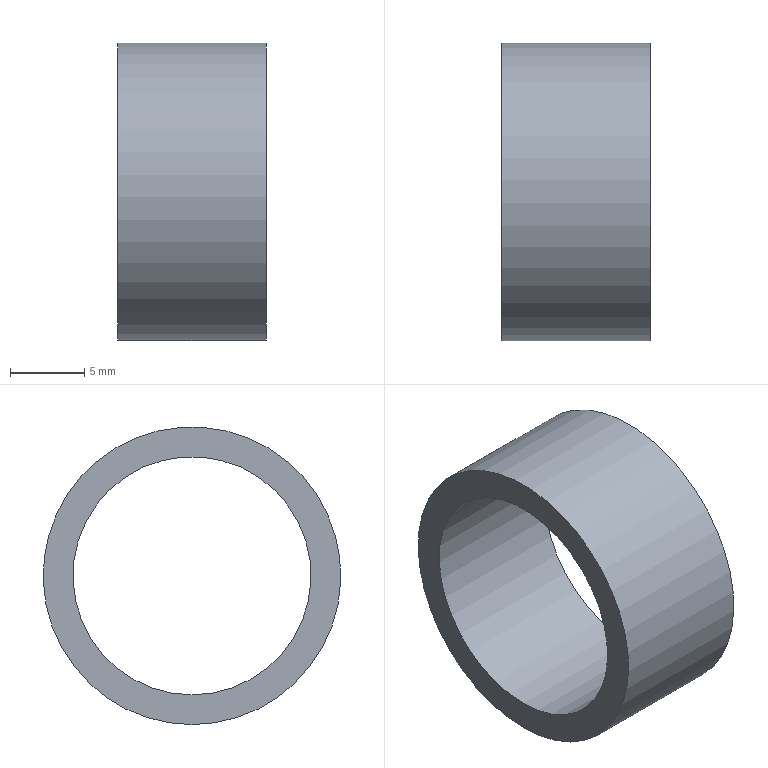Component | NX | BUSHING | 1 solid | 4 faces | box 10 x 20 x 20 mm | volume 1131 mm3 | cylinder 2 | plane 2 | commonest cylinder face diameters 20 x1 16 x1
STEP:
#1=CARTESIAN_POINT('',(0.,0.,0.));
#2=DIRECTION('',(0.,0.,1.));
#3=DIRECTION('',(1.,0.,0.));
#4=AXIS2_PLACEMENT_3D('',#1,#2,#3);
#5=CARTESIAN_POINT('',(25.,110.,-100.));
#6=VERTEX_POINT('',#5);
#7=CARTESIAN_POINT('',(25.,110.,-90.));
#8=DIRECTION('',(1.,0.,0.));
#9=DIRECTION('',(0.,0.,-1.));
#10=AXIS2_PLACEMENT_3D('',#7,#8,#9);
#11=CIRCLE('',#10,10.);
#12=CARTESIAN_POINT('',(25.,110.,-90.));
#13=DIRECTION('',(1.,0.,0.));
#14=DIRECTION('',(0.,0.,-1.));
#15=AXIS2_PLACEMENT_3D('',#12,#13,#14);
#16=CYLINDRICAL_SURFACE('',#15,10.);
#17=CARTESIAN_POINT('',(0.,0.));
#18=DIRECTION('',(1.,0.));
#19=VECTOR('',#18,1.);
#20=LINE('',#17,#19);
#21=(GEOMETRIC_REPRESENTATION_CONTEXT(2)PARAMETRIC_REPRESENTATION_CONTEXT()REPRESENTATION_CONTEXT('',''));
#22=DEFINITIONAL_REPRESENTATION('',(#20),#21);
#23=PCURVE('',#16,#22);
#24=CARTESIAN_POINT('',(25.,110.,-90.));
#25=DIRECTION('',(1.,0.,0.));
#26=DIRECTION('',(0.,0.,-1.));
#27=AXIS2_PLACEMENT_3D('',#24,#25,#26);
#28=PLANE('',#27);
#29=CARTESIAN_POINT('',(0.,0.));
#30=DIRECTION('',(1.,0.));
#31=AXIS2_PLACEMENT_2D('',#29,#30);
#32=CIRCLE('',#31,10.);
#33=(GEOMETRIC_REPRESENTATION_CONTEXT(2)PARAMETRIC_REPRESENTATION_CONTEXT()REPRESENTATION_CONTEXT('',''));
#34=DEFINITIONAL_REPRESENTATION('',(#32),#33);
#35=PCURVE('',#28,#34);
#36=SURFACE_CURVE('',#11,(#23,#35),.PCURVE_S1.);
#37=EDGE_CURVE('',#6,#6,#36,.T.);
#38=ORIENTED_EDGE('',*,*,#37,.T.);
#39=CARTESIAN_POINT('',(35.,110.,-100.));
#40=VERTEX_POINT('',#39);
#41=CARTESIAN_POINT('',(25.,110.,-100.));
#42=CARTESIAN_POINT('',(35.,110.,-100.));
#43=B_SPLINE_CURVE_WITH_KNOTS('',1,(#41,#42),.UNSPECIFIED.,.F.,.F.,(2,2),(0.,10.),.PIECEWISE_BEZIER_KNOTS.);
#44=CARTESIAN_POINT('',(6.283,0.));
#45=DIRECTION('',(0.,1.));
#46=VECTOR('',#45,1.);
#47=LINE('',#44,#46);
#48=(GEOMETRIC_REPRESENTATION_CONTEXT(2)PARAMETRIC_REPRESENTATION_CONTEXT()REPRESENTATION_CONTEXT('',''));
#49=DEFINITIONAL_REPRESENTATION('',(#47),#48);
#50=PCURVE('',#16,#49);
#51=CARTESIAN_POINT('',(0.,0.));
#52=DIRECTION('',(0.,1.));
#53=VECTOR('',#52,1.);
#54=LINE('',#51,#53);
#55=(GEOMETRIC_REPRESENTATION_CONTEXT(2)PARAMETRIC_REPRESENTATION_CONTEXT()REPRESENTATION_CONTEXT('',''));
#56=DEFINITIONAL_REPRESENTATION('',(#54),#55);
#57=PCURVE('',#16,#56);
#58=SEAM_CURVE('',#43,(#50,#57),.PCURVE_S1.);
#59=EDGE_CURVE('',#6,#40,#58,.T.);
#60=ORIENTED_EDGE('',*,*,#59,.T.);
#61=CARTESIAN_POINT('',(35.,110.,-90.));
#62=DIRECTION('',(1.,0.,0.));
#63=DIRECTION('',(0.,0.,-1.));
#64=AXIS2_PLACEMENT_3D('',#61,#62,#63);
#65=CIRCLE('',#64,10.);
#66=CARTESIAN_POINT('',(0.,10.));
#67=DIRECTION('',(1.,0.));
#68=VECTOR('',#67,1.);
#69=LINE('',#66,#68);
#70=(GEOMETRIC_REPRESENTATION_CONTEXT(2)PARAMETRIC_REPRESENTATION_CONTEXT()REPRESENTATION_CONTEXT('',''));
#71=DEFINITIONAL_REPRESENTATION('',(#69),#70);
#72=PCURVE('',#16,#71);
#73=CARTESIAN_POINT('',(35.,110.,-90.));
#74=DIRECTION('',(1.,0.,0.));
#75=DIRECTION('',(0.,0.,-1.));
#76=AXIS2_PLACEMENT_3D('',#73,#74,#75);
#77=PLANE('',#76);
#78=CARTESIAN_POINT('',(0.,0.));
#79=DIRECTION('',(1.,0.));
#80=AXIS2_PLACEMENT_2D('',#78,#79);
#81=CIRCLE('',#80,10.);
#82=(GEOMETRIC_REPRESENTATION_CONTEXT(2)PARAMETRIC_REPRESENTATION_CONTEXT()REPRESENTATION_CONTEXT('',''));
#83=DEFINITIONAL_REPRESENTATION('',(#81),#82);
#84=PCURVE('',#77,#83);
#85=SURFACE_CURVE('',#65,(#72,#84),.PCURVE_S1.);
#86=EDGE_CURVE('',#40,#40,#85,.T.);
#87=ORIENTED_EDGE('',*,*,#86,.F.);
#88=ORIENTED_EDGE('',*,*,#59,.F.);
#89=EDGE_LOOP('',(#38,#60,#87,#88));
#90=FACE_BOUND('',#89,.T.);
#91=ADVANCED_FACE('',(#90),#16,.T.);
#92=CARTESIAN_POINT('',(25.,110.,-98.));
#93=VERTEX_POINT('',#92);
#94=CARTESIAN_POINT('',(25.,110.,-90.));
#95=DIRECTION('',(1.,0.,0.));
#96=DIRECTION('',(0.,0.,-1.));
#97=AXIS2_PLACEMENT_3D('',#94,#95,#96);
#98=CIRCLE('',#97,8.);
#99=CARTESIAN_POINT('',(25.,110.,-90.));
#100=DIRECTION('',(1.,0.,0.));
#101=DIRECTION('',(0.,0.,-1.));
#102=AXIS2_PLACEMENT_3D('',#99,#100,#101);
#103=CYLINDRICAL_SURFACE('',#102,8.);
#104=CARTESIAN_POINT('',(0.,0.));
#105=DIRECTION('',(1.,0.));
#106=VECTOR('',#105,1.);
#107=LINE('',#104,#106);
#108=(GEOMETRIC_REPRESENTATION_CONTEXT(2)PARAMETRIC_REPRESENTATION_CONTEXT()REPRESENTATION_CONTEXT('',''));
#109=DEFINITIONAL_REPRESENTATION('',(#107),#108);
#110=PCURVE('',#103,#109);
#111=CARTESIAN_POINT('',(0.,0.));
#112=DIRECTION('',(1.,0.));
#113=AXIS2_PLACEMENT_2D('',#111,#112);
#114=CIRCLE('',#113,8.);
#115=(GEOMETRIC_REPRESENTATION_CONTEXT(2)PARAMETRIC_REPRESENTATION_CONTEXT()REPRESENTATION_CONTEXT('',''));
#116=DEFINITIONAL_REPRESENTATION('',(#114),#115);
#117=PCURVE('',#28,#116);
#118=SURFACE_CURVE('',#98,(#110,#117),.PCURVE_S1.);
#119=EDGE_CURVE('',#93,#93,#118,.T.);
#120=ORIENTED_EDGE('',*,*,#119,.T.);
#121=CARTESIAN_POINT('',(35.,110.,-98.));
#122=VERTEX_POINT('',#121);
#123=CARTESIAN_POINT('',(25.,110.,-98.));
#124=CARTESIAN_POINT('',(35.,110.,-98.));
#125=B_SPLINE_CURVE_WITH_KNOTS('',1,(#123,#124),.UNSPECIFIED.,.F.,.F.,(2,2),(0.,10.),.PIECEWISE_BEZIER_KNOTS.);
#126=CARTESIAN_POINT('',(6.283,0.));
#127=DIRECTION('',(0.,1.));
#128=VECTOR('',#127,1.);
#129=LINE('',#126,#128);
#130=(GEOMETRIC_REPRESENTATION_CONTEXT(2)PARAMETRIC_REPRESENTATION_CONTEXT()REPRESENTATION_CONTEXT('',''));
#131=DEFINITIONAL_REPRESENTATION('',(#129),#130);
#132=PCURVE('',#103,#131);
#133=CARTESIAN_POINT('',(0.,0.));
#134=DIRECTION('',(0.,1.));
#135=VECTOR('',#134,1.);
#136=LINE('',#133,#135);
#137=(GEOMETRIC_REPRESENTATION_CONTEXT(2)PARAMETRIC_REPRESENTATION_CONTEXT()REPRESENTATION_CONTEXT('',''));
#138=DEFINITIONAL_REPRESENTATION('',(#136),#137);
#139=PCURVE('',#103,#138);
#140=SEAM_CURVE('',#125,(#132,#139),.PCURVE_S1.);
#141=EDGE_CURVE('',#93,#122,#140,.T.);
#142=ORIENTED_EDGE('',*,*,#141,.T.);
#143=CARTESIAN_POINT('',(35.,110.,-90.));
#144=DIRECTION('',(1.,0.,0.));
#145=DIRECTION('',(0.,0.,-1.));
#146=AXIS2_PLACEMENT_3D('',#143,#144,#145);
#147=CIRCLE('',#146,8.);
#148=CARTESIAN_POINT('',(0.,10.));
#149=DIRECTION('',(1.,0.));
#150=VECTOR('',#149,1.);
#151=LINE('',#148,#150);
#152=(GEOMETRIC_REPRESENTATION_CONTEXT(2)PARAMETRIC_REPRESENTATION_CONTEXT()REPRESENTATION_CONTEXT('',''));
#153=DEFINITIONAL_REPRESENTATION('',(#151),#152);
#154=PCURVE('',#103,#153);
#155=CARTESIAN_POINT('',(0.,0.));
#156=DIRECTION('',(1.,0.));
#157=AXIS2_PLACEMENT_2D('',#155,#156);
#158=CIRCLE('',#157,8.);
#159=(GEOMETRIC_REPRESENTATION_CONTEXT(2)PARAMETRIC_REPRESENTATION_CONTEXT()REPRESENTATION_CONTEXT('',''));
#160=DEFINITIONAL_REPRESENTATION('',(#158),#159);
#161=PCURVE('',#77,#160);
#162=SURFACE_CURVE('',#147,(#154,#161),.PCURVE_S1.);
#163=EDGE_CURVE('',#122,#122,#162,.T.);
#164=ORIENTED_EDGE('',*,*,#163,.F.);
#165=ORIENTED_EDGE('',*,*,#141,.F.);
#166=EDGE_LOOP('',(#120,#142,#164,#165));
#167=FACE_BOUND('',#166,.F.);
#168=ADVANCED_FACE('',(#167),#103,.F.);
#169=ORIENTED_EDGE('',*,*,#37,.F.);
#170=EDGE_LOOP('',(#169));
#171=FACE_BOUND('',#170,.T.);
#172=ORIENTED_EDGE('',*,*,#119,.T.);
#173=EDGE_LOOP('',(#172));
#174=FACE_BOUND('',#173,.T.);
#175=ADVANCED_FACE('',(#171,#174),#28,.F.);
#176=ORIENTED_EDGE('',*,*,#86,.T.);
#177=EDGE_LOOP('',(#176));
#178=FACE_BOUND('',#177,.T.);
#179=ORIENTED_EDGE('',*,*,#163,.F.);
#180=EDGE_LOOP('',(#179));
#181=FACE_BOUND('',#180,.T.);
#182=ADVANCED_FACE('',(#178,#181),#77,.T.);
#183=CLOSED_SHELL('',(#91,#168,#175,#182));
#184=MANIFOLD_SOLID_BREP('',#183);
#185=(LENGTH_UNIT()NAMED_UNIT(*)SI_UNIT(.MILLI.,.METRE.));
#186=UNCERTAINTY_MEASURE_WITH_UNIT(LENGTH_MEASURE(0.00001),#185,'','');
#187=(NAMED_UNIT(*)PLANE_ANGLE_UNIT()SI_UNIT($,.RADIAN.));
#188=(NAMED_UNIT(*)SI_UNIT($,.STERADIAN.)SOLID_ANGLE_UNIT());
#189=(GEOMETRIC_REPRESENTATION_CONTEXT(3)GLOBAL_UNCERTAINTY_ASSIGNED_CONTEXT((#186))GLOBAL_UNIT_ASSIGNED_CONTEXT((#185,#187,#188))REPRESENTATION_CONTEXT('',''));
#190=ADVANCED_BREP_SHAPE_REPRESENTATION('',(#4,#184),#189);